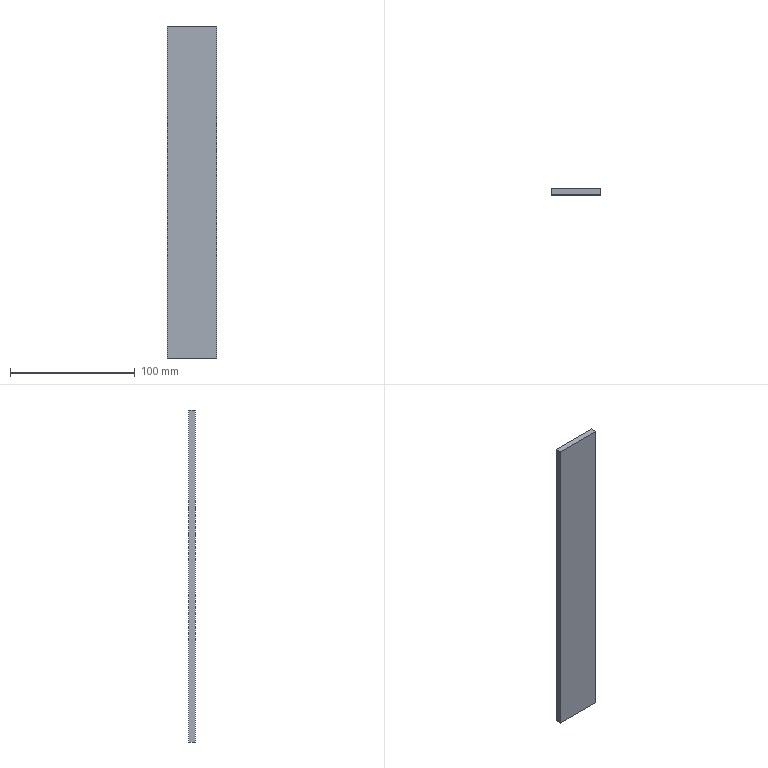Component | SolidWorks | LD101-02--Q1069-Q1-2-3 | 1 solid | 6 faces | box 40 x 5 x 266 mm | volume 53200 mm3 | plane 6 | material Nylon1010
build123d program:
from build123d import *

# Parameters (mm, degrees)
SKETCH1_W           = 266
SKETCH1_H           = 40
BOSS_EXTRUDE1_DEPTH = 2.5


with BuildPart() as part:
    # Sketch1 → Boss-Extrude1 (new, symmetric)
    with BuildSketch(Plane(origin=(0, 0, 0), x_dir=(1, 0, 0), z_dir=(0, 1, 0))):
        Rectangle(SKETCH1_W, SKETCH1_H)
    extrude(amount=BOSS_EXTRUDE1_DEPTH, both=True)


solid = part.part

# Placed as in the assembly
solid = solid.moved(Location((49.71, -151.397, 146.257), (0, 90, 0)))
STEP:
#1=COLOUR_RGB('',0.7922,0.8196,0.9333);
#2=FILL_AREA_STYLE_COLOUR('',#1);
#3=FILL_AREA_STYLE('',(#2));
#4=SURFACE_STYLE_FILL_AREA(#3);
#5=SURFACE_SIDE_STYLE('',(#4));
#6=SURFACE_STYLE_USAGE(.BOTH.,#5);
#7=PRESENTATION_STYLE_ASSIGNMENT((#6));
#8=CARTESIAN_POINT('',(2.744,-5.862,10.994));
#9=VERTEX_POINT('',#8);
#10=CARTESIAN_POINT('',(1.17,-5.862,10.994));
#11=VERTEX_POINT('',#10);
#12=CARTESIAN_POINT('',(2.744,-5.862,10.994));
#13=DIRECTION('',(-1.,-0.,0.));
#14=VECTOR('',#13,39.37);
#15=LINE('',#12,#14);
#16=EDGE_CURVE('',#9,#11,#15,.T.);
#17=ORIENTED_EDGE('',*,*,#16,.T.);
#18=CARTESIAN_POINT('',(1.17,-6.059,10.994));
#19=VERTEX_POINT('',#18);
#20=CARTESIAN_POINT('',(1.17,-6.059,10.994));
#21=DIRECTION('',(0.,1.,-0.));
#22=VECTOR('',#21,39.37);
#23=LINE('',#20,#22);
#24=EDGE_CURVE('',#19,#11,#23,.T.);
#25=ORIENTED_EDGE('',*,*,#24,.F.);
#26=CARTESIAN_POINT('',(2.744,-6.059,10.994));
#27=VERTEX_POINT('',#26);
#28=CARTESIAN_POINT('',(2.744,-6.059,10.994));
#29=DIRECTION('',(-1.,-0.,0.));
#30=VECTOR('',#29,39.37);
#31=LINE('',#28,#30);
#32=EDGE_CURVE('',#27,#19,#31,.T.);
#33=ORIENTED_EDGE('',*,*,#32,.F.);
#34=CARTESIAN_POINT('',(2.744,-6.059,10.994));
#35=DIRECTION('',(0.,1.,-0.));
#36=VECTOR('',#35,39.37);
#37=LINE('',#34,#36);
#38=EDGE_CURVE('',#27,#9,#37,.T.);
#39=ORIENTED_EDGE('',*,*,#38,.T.);
#40=EDGE_LOOP('',(#17,#25,#33,#39));
#41=FACE_OUTER_BOUND('',#40,.T.);
#42=CARTESIAN_POINT('',(2.744,-6.059,10.994));
#43=DIRECTION('',(-0.,-0.,-1.));
#44=DIRECTION('',(1.,0.,-0.));
#45=AXIS2_PLACEMENT_3D('',#42,#43,#44);
#46=PLANE('',#45);
#47=ADVANCED_FACE('',(#41),#46,.F.);
#48=CARTESIAN_POINT('',(1.17,-5.862,0.5219));
#49=VERTEX_POINT('',#48);
#50=CARTESIAN_POINT('',(1.17,-5.862,0.5219));
#51=DIRECTION('',(-0.,-0.,-1.));
#52=VECTOR('',#51,39.37);
#53=LINE('',#50,#52);
#54=EDGE_CURVE('',#11,#49,#53,.T.);
#55=ORIENTED_EDGE('',*,*,#54,.T.);
#56=CARTESIAN_POINT('',(1.17,-6.059,0.5219));
#57=VERTEX_POINT('',#56);
#58=CARTESIAN_POINT('',(1.17,-6.059,0.5219));
#59=DIRECTION('',(0.,1.,-0.));
#60=VECTOR('',#59,39.37);
#61=LINE('',#58,#60);
#62=EDGE_CURVE('',#57,#49,#61,.T.);
#63=ORIENTED_EDGE('',*,*,#62,.F.);
#64=CARTESIAN_POINT('',(1.17,-6.059,0.5219));
#65=DIRECTION('',(-0.,-0.,-1.));
#66=VECTOR('',#65,39.37);
#67=LINE('',#64,#66);
#68=EDGE_CURVE('',#19,#57,#67,.T.);
#69=ORIENTED_EDGE('',*,*,#68,.F.);
#70=ORIENTED_EDGE('',*,*,#24,.T.);
#71=EDGE_LOOP('',(#55,#63,#69,#70));
#72=FACE_OUTER_BOUND('',#71,.T.);
#73=CARTESIAN_POINT('',(1.17,-6.059,0.5219));
#74=DIRECTION('',(1.,0.,-0.));
#75=DIRECTION('',(0.,0.,1.));
#76=AXIS2_PLACEMENT_3D('',#73,#74,#75);
#77=PLANE('',#76);
#78=ADVANCED_FACE('',(#72),#77,.F.);
#79=CARTESIAN_POINT('',(2.744,-5.862,0.5219));
#80=VERTEX_POINT('',#79);
#81=CARTESIAN_POINT('',(2.744,-5.862,0.5219));
#82=DIRECTION('',(1.,0.,-0.));
#83=VECTOR('',#82,39.37);
#84=LINE('',#81,#83);
#85=EDGE_CURVE('',#49,#80,#84,.T.);
#86=ORIENTED_EDGE('',*,*,#85,.T.);
#87=CARTESIAN_POINT('',(2.744,-6.059,0.5219));
#88=VERTEX_POINT('',#87);
#89=CARTESIAN_POINT('',(2.744,-6.059,0.5219));
#90=DIRECTION('',(0.,1.,-0.));
#91=VECTOR('',#90,39.37);
#92=LINE('',#89,#91);
#93=EDGE_CURVE('',#88,#80,#92,.T.);
#94=ORIENTED_EDGE('',*,*,#93,.F.);
#95=CARTESIAN_POINT('',(2.744,-6.059,0.5219));
#96=DIRECTION('',(1.,0.,-0.));
#97=VECTOR('',#96,39.37);
#98=LINE('',#95,#97);
#99=EDGE_CURVE('',#57,#88,#98,.T.);
#100=ORIENTED_EDGE('',*,*,#99,.F.);
#101=ORIENTED_EDGE('',*,*,#62,.T.);
#102=EDGE_LOOP('',(#86,#94,#100,#101));
#103=FACE_OUTER_BOUND('',#102,.T.);
#104=CARTESIAN_POINT('',(2.744,-6.059,0.5219));
#105=DIRECTION('',(0.,0.,1.));
#106=DIRECTION('',(-1.,-0.,0.));
#107=AXIS2_PLACEMENT_3D('',#104,#105,#106);
#108=PLANE('',#107);
#109=ADVANCED_FACE('',(#103),#108,.F.);
#110=CARTESIAN_POINT('',(2.744,-5.862,0.5219));
#111=DIRECTION('',(0.,0.,1.));
#112=VECTOR('',#111,39.37);
#113=LINE('',#110,#112);
#114=EDGE_CURVE('',#80,#9,#113,.T.);
#115=ORIENTED_EDGE('',*,*,#114,.T.);
#116=ORIENTED_EDGE('',*,*,#38,.F.);
#117=CARTESIAN_POINT('',(2.744,-6.059,0.5219));
#118=DIRECTION('',(0.,0.,1.));
#119=VECTOR('',#118,39.37);
#120=LINE('',#117,#119);
#121=EDGE_CURVE('',#88,#27,#120,.T.);
#122=ORIENTED_EDGE('',*,*,#121,.F.);
#123=ORIENTED_EDGE('',*,*,#93,.T.);
#124=EDGE_LOOP('',(#115,#116,#122,#123));
#125=FACE_OUTER_BOUND('',#124,.T.);
#126=CARTESIAN_POINT('',(2.744,-6.059,0.5219));
#127=DIRECTION('',(-1.,-0.,0.));
#128=DIRECTION('',(-0.,-0.,-1.));
#129=AXIS2_PLACEMENT_3D('',#126,#127,#128);
#130=PLANE('',#129);
#131=ADVANCED_FACE('',(#125),#130,.F.);
#132=ORIENTED_EDGE('',*,*,#32,.T.);
#133=ORIENTED_EDGE('',*,*,#68,.T.);
#134=ORIENTED_EDGE('',*,*,#99,.T.);
#135=ORIENTED_EDGE('',*,*,#121,.T.);
#136=EDGE_LOOP('',(#132,#133,#134,#135));
#137=FACE_OUTER_BOUND('',#136,.T.);
#138=CARTESIAN_POINT('',(1.957,-6.059,5.758));
#139=DIRECTION('',(-0.,1.,-0.));
#140=DIRECTION('',(-1.,-0.,0.));
#141=AXIS2_PLACEMENT_3D('',#138,#139,#140);
#142=PLANE('',#141);
#143=ADVANCED_FACE('',(#137),#142,.F.);
#144=ORIENTED_EDGE('',*,*,#16,.F.);
#145=ORIENTED_EDGE('',*,*,#114,.F.);
#146=ORIENTED_EDGE('',*,*,#85,.F.);
#147=ORIENTED_EDGE('',*,*,#54,.F.);
#148=EDGE_LOOP('',(#144,#145,#146,#147));
#149=FACE_OUTER_BOUND('',#148,.T.);
#150=CARTESIAN_POINT('',(1.957,-5.862,5.758));
#151=DIRECTION('',(-0.,1.,-0.));
#152=DIRECTION('',(-1.,-0.,0.));
#153=AXIS2_PLACEMENT_3D('',#150,#151,#152);
#154=PLANE('',#153);
#155=ADVANCED_FACE('',(#149),#154,.T.);
#156=CLOSED_SHELL('',(#47,#78,#109,#131,#143,#155));
#157=MANIFOLD_SOLID_BREP('',#156);
#158=STYLED_ITEM('',(#7),#157);
#159=PRESENTATION_LAYER_ASSIGNMENT('','',(#158));
#160=(LENGTH_UNIT()NAMED_UNIT(*)SI_UNIT($,.METRE.));
#161=LENGTH_MEASURE_WITH_UNIT(LENGTH_MEASURE(0.0254),#160);
#162=DIMENSIONAL_EXPONENTS(1.,0.,0.,0.,0.,0.,0.);
#163=(CONVERSION_BASED_UNIT('',#161)LENGTH_UNIT()NAMED_UNIT(#162));
#164=UNCERTAINTY_MEASURE_WITH_UNIT(LENGTH_MEASURE(0.00001),#163,'','');
#165=(NAMED_UNIT(*)PLANE_ANGLE_UNIT()SI_UNIT($,.RADIAN.));
#166=(NAMED_UNIT(*)SI_UNIT($,.STERADIAN.)SOLID_ANGLE_UNIT());
#167=(GEOMETRIC_REPRESENTATION_CONTEXT(3)GLOBAL_UNCERTAINTY_ASSIGNED_CONTEXT((#164))GLOBAL_UNIT_ASSIGNED_CONTEXT((#163,#165,#166))REPRESENTATION_CONTEXT('',''));
#168=MECHANICAL_DESIGN_GEOMETRIC_PRESENTATION_REPRESENTATION('',(#158),#167);
#169=CARTESIAN_POINT('',(0.,0.,0.));
#170=DIRECTION('',(0.,0.,1.));
#171=DIRECTION('',(1.,0.,0.));
#172=AXIS2_PLACEMENT_3D('',#169,#170,#171);
#173=(LENGTH_UNIT()NAMED_UNIT(*)SI_UNIT($,.METRE.));
#174=LENGTH_MEASURE_WITH_UNIT(LENGTH_MEASURE(0.0254),#173);
#175=DIMENSIONAL_EXPONENTS(1.,0.,0.,0.,0.,0.,0.);
#176=(CONVERSION_BASED_UNIT('',#174)LENGTH_UNIT()NAMED_UNIT(#175));
#177=UNCERTAINTY_MEASURE_WITH_UNIT(LENGTH_MEASURE(0.00001),#176,'','');
#178=(NAMED_UNIT(*)PLANE_ANGLE_UNIT()SI_UNIT($,.RADIAN.));
#179=(NAMED_UNIT(*)SI_UNIT($,.STERADIAN.)SOLID_ANGLE_UNIT());
#180=(GEOMETRIC_REPRESENTATION_CONTEXT(3)GLOBAL_UNCERTAINTY_ASSIGNED_CONTEXT((#177))GLOBAL_UNIT_ASSIGNED_CONTEXT((#176,#178,#179))REPRESENTATION_CONTEXT('',''));
#181=ADVANCED_BREP_SHAPE_REPRESENTATION('',(#157,#172),#180);